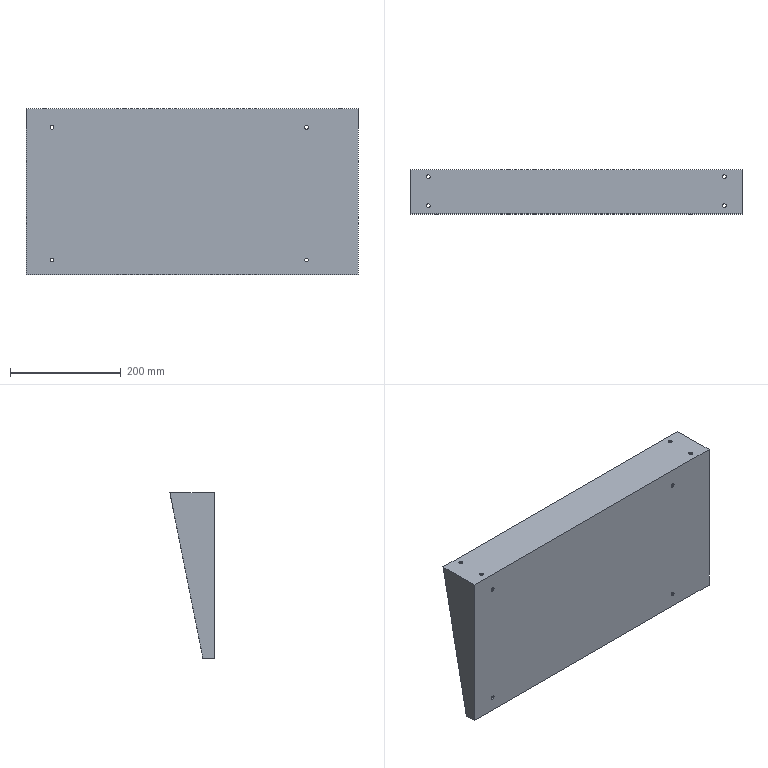Component | SolidWorks | OilTankBracket-1 | 1 solid | 26 faces | box 600 x 80 x 300 mm | volume 760356 mm3 | cylinder 16 | plane 10 | commonest cylinder face diameters 7 x16
build123d program:
from build123d import *

# Parameters (mm, degrees)
BOSS_EXTRUDE1_DEPTH = 600
SHELL1_T            = -3
SKETCH3_R           = 3.5
CUT_EXTRUDE1_DEPTH  = 3
LPATTERN1_COUNT     = 2
LPATTERN1_PITCH     = 535
SKETCH4_R           = 3.5
CUT_EXTRUDE2_DEPTH  = 3


with BuildPart() as part:
    # Sketch2 → Boss-Extrude1 (new body)
    with BuildSketch(Plane.XY):
        Polygon((17.897, -71.247), (17.897, 8.753), (317.897, 8.753), (317.897, -11.247), align=None)
    extrude(amount=BOSS_EXTRUDE1_DEPTH)

    # Shell1
    shell1_openings = [part.faces().sort_by_distance(p)[0] for p in [
        (317.897, -1.247, 300),
        (167.897, -41.247, 300),
    ]]
    offset(amount=SHELL1_T, openings=shell1_openings, kind=Kind.INTERSECTION)

    # Sketch3 → Cut-Extrude1 (cut)
    with BuildSketch(Plane(origin=(20.897, 0, 0), x_dir=(0, 0, -1), z_dir=(1, 0, 0))):
        with Locations((-567, -6.247)):
            Circle(SKETCH3_R)
        with Locations((-567, -58.647)):
            Circle(SKETCH3_R)
    cut_extrude1 = extrude(amount=-CUT_EXTRUDE1_DEPTH, mode=Mode.SUBTRACT)

    # LPattern1: Cut-Extrude1 ×2
    with Locations(*[(0, 0, -i * LPATTERN1_PITCH) for i in range(1, LPATTERN1_COUNT)]):
        add(cut_extrude1, mode=Mode.SUBTRACT)

    # Sketch4 → Cut-Extrude2 (cut)
    with BuildSketch(Plane(origin=(0, 5.753, 0), x_dir=(-1, 0, 0), z_dir=(0, -1, 0))):
        with Locations(Location((-290.897, -553, 0), (0, 0, 90))):
            Circle(SKETCH4_R)
        with Locations(Location((-50.897, -553, 0), (0, 0, 90))):
            Circle(SKETCH4_R)
        with Locations(Location((-290.897, -93, 0), (0, 0, 90))):
            Circle(SKETCH4_R)
        with Locations(Location((-50.897, -93, 0), (0, 0, 90))):
            Circle(SKETCH4_R)
    extrude(amount=-CUT_EXTRUDE2_DEPTH, mode=Mode.SUBTRACT)


solid = part.part

# Placed as in the assembly
solid = solid.moved(Location((508.45, -702.681, -350.622), (180, -90, 0)))
STEP:
#1=CARTESIAN_POINT('',(16.219,-28.009,-15.808));
#2=VERTEX_POINT('',#1);
#3=CARTESIAN_POINT('',(16.494,-28.009,-15.808));
#4=VERTEX_POINT('',#3);
#5=CARTESIAN_POINT('',(16.356,-28.009,-15.808));
#6=DIRECTION('',(0.,1.,0.));
#7=DIRECTION('',(1.,0.,0.));
#8=AXIS2_PLACEMENT_3D('',#5,#6,#7);
#9=CIRCLE('',#8,0.1378);
#10=EDGE_CURVE('',#2,#4,#9,.T.);
#11=ORIENTED_EDGE('',*,*,#10,.F.);
#12=CARTESIAN_POINT('',(16.219,-27.891,-15.808));
#13=VERTEX_POINT('',#12);
#14=CARTESIAN_POINT('',(16.219,-28.009,-15.808));
#15=DIRECTION('',(0.,1.,0.));
#16=VECTOR('',#15,39.37);
#17=LINE('',#14,#16);
#18=EDGE_CURVE('',#2,#13,#17,.T.);
#19=ORIENTED_EDGE('',*,*,#18,.T.);
#20=CARTESIAN_POINT('',(16.494,-27.891,-15.808));
#21=VERTEX_POINT('',#20);
#22=CARTESIAN_POINT('',(16.356,-27.891,-15.808));
#23=DIRECTION('',(0.,1.,0.));
#24=DIRECTION('',(1.,0.,0.));
#25=AXIS2_PLACEMENT_3D('',#22,#23,#24);
#26=CIRCLE('',#25,0.1378);
#27=EDGE_CURVE('',#13,#21,#26,.T.);
#28=ORIENTED_EDGE('',*,*,#27,.T.);
#29=CARTESIAN_POINT('',(16.494,-28.009,-15.808));
#30=DIRECTION('',(0.,1.,0.));
#31=VECTOR('',#30,39.37);
#32=LINE('',#29,#31);
#33=EDGE_CURVE('',#4,#21,#32,.T.);
#34=ORIENTED_EDGE('',*,*,#33,.F.);
#35=EDGE_LOOP('',(#11,#19,#28,#34));
#36=FACE_OUTER_BOUND('',#35,.T.);
#37=CARTESIAN_POINT('',(16.356,-28.009,-15.808));
#38=DIRECTION('',(0.,1.,0.));
#39=DIRECTION('',(1.,0.,0.));
#40=AXIS2_PLACEMENT_3D('',#37,#38,#39);
#41=CYLINDRICAL_SURFACE('',#40,0.1378);
#42=ADVANCED_FACE('',(#36),#41,.F.);
#43=CARTESIAN_POINT('',(16.219,-28.009,-25.257));
#44=VERTEX_POINT('',#43);
#45=CARTESIAN_POINT('',(16.494,-28.009,-25.257));
#46=VERTEX_POINT('',#45);
#47=CARTESIAN_POINT('',(16.356,-28.009,-25.257));
#48=DIRECTION('',(0.,1.,0.));
#49=DIRECTION('',(1.,0.,0.));
#50=AXIS2_PLACEMENT_3D('',#47,#48,#49);
#51=CIRCLE('',#50,0.1378);
#52=EDGE_CURVE('',#44,#46,#51,.T.);
#53=ORIENTED_EDGE('',*,*,#52,.F.);
#54=CARTESIAN_POINT('',(16.219,-27.891,-25.257));
#55=VERTEX_POINT('',#54);
#56=CARTESIAN_POINT('',(16.219,-28.009,-25.257));
#57=DIRECTION('',(0.,1.,0.));
#58=VECTOR('',#57,39.37);
#59=LINE('',#56,#58);
#60=EDGE_CURVE('',#44,#55,#59,.T.);
#61=ORIENTED_EDGE('',*,*,#60,.T.);
#62=CARTESIAN_POINT('',(16.494,-27.891,-25.257));
#63=VERTEX_POINT('',#62);
#64=CARTESIAN_POINT('',(16.356,-27.891,-25.257));
#65=DIRECTION('',(0.,1.,0.));
#66=DIRECTION('',(1.,0.,0.));
#67=AXIS2_PLACEMENT_3D('',#64,#65,#66);
#68=CIRCLE('',#67,0.1378);
#69=EDGE_CURVE('',#55,#63,#68,.T.);
#70=ORIENTED_EDGE('',*,*,#69,.T.);
#71=CARTESIAN_POINT('',(16.494,-28.009,-25.257));
#72=DIRECTION('',(0.,1.,0.));
#73=VECTOR('',#72,39.37);
#74=LINE('',#71,#73);
#75=EDGE_CURVE('',#46,#63,#74,.T.);
#76=ORIENTED_EDGE('',*,*,#75,.F.);
#77=EDGE_LOOP('',(#53,#61,#70,#76));
#78=FACE_OUTER_BOUND('',#77,.T.);
#79=CARTESIAN_POINT('',(16.356,-28.009,-25.257));
#80=DIRECTION('',(0.,1.,0.));
#81=DIRECTION('',(1.,0.,0.));
#82=AXIS2_PLACEMENT_3D('',#79,#80,#81);
#83=CYLINDRICAL_SURFACE('',#82,0.1378);
#84=ADVANCED_FACE('',(#78),#83,.F.);
#85=CARTESIAN_POINT('',(-1.892,-28.009,-15.808));
#86=VERTEX_POINT('',#85);
#87=CARTESIAN_POINT('',(-1.616,-28.009,-15.808));
#88=VERTEX_POINT('',#87);
#89=CARTESIAN_POINT('',(-1.754,-28.009,-15.808));
#90=DIRECTION('',(0.,1.,0.));
#91=DIRECTION('',(1.,0.,0.));
#92=AXIS2_PLACEMENT_3D('',#89,#90,#91);
#93=CIRCLE('',#92,0.1378);
#94=EDGE_CURVE('',#86,#88,#93,.T.);
#95=ORIENTED_EDGE('',*,*,#94,.F.);
#96=CARTESIAN_POINT('',(-1.892,-27.891,-15.808));
#97=VERTEX_POINT('',#96);
#98=CARTESIAN_POINT('',(-1.892,-28.009,-15.808));
#99=DIRECTION('',(0.,1.,0.));
#100=VECTOR('',#99,39.37);
#101=LINE('',#98,#100);
#102=EDGE_CURVE('',#86,#97,#101,.T.);
#103=ORIENTED_EDGE('',*,*,#102,.T.);
#104=CARTESIAN_POINT('',(-1.616,-27.891,-15.808));
#105=VERTEX_POINT('',#104);
#106=CARTESIAN_POINT('',(-1.754,-27.891,-15.808));
#107=DIRECTION('',(0.,1.,0.));
#108=DIRECTION('',(1.,0.,0.));
#109=AXIS2_PLACEMENT_3D('',#106,#107,#108);
#110=CIRCLE('',#109,0.1378);
#111=EDGE_CURVE('',#97,#105,#110,.T.);
#112=ORIENTED_EDGE('',*,*,#111,.T.);
#113=CARTESIAN_POINT('',(-1.616,-28.009,-15.808));
#114=DIRECTION('',(0.,1.,0.));
#115=VECTOR('',#114,39.37);
#116=LINE('',#113,#115);
#117=EDGE_CURVE('',#88,#105,#116,.T.);
#118=ORIENTED_EDGE('',*,*,#117,.F.);
#119=EDGE_LOOP('',(#95,#103,#112,#118));
#120=FACE_OUTER_BOUND('',#119,.T.);
#121=CARTESIAN_POINT('',(-1.754,-28.009,-15.808));
#122=DIRECTION('',(0.,1.,0.));
#123=DIRECTION('',(1.,0.,0.));
#124=AXIS2_PLACEMENT_3D('',#121,#122,#123);
#125=CYLINDRICAL_SURFACE('',#124,0.1378);
#126=ADVANCED_FACE('',(#120),#125,.F.);
#127=CARTESIAN_POINT('',(-1.892,-28.009,-25.257));
#128=VERTEX_POINT('',#127);
#129=CARTESIAN_POINT('',(-1.616,-28.009,-25.257));
#130=VERTEX_POINT('',#129);
#131=CARTESIAN_POINT('',(-1.754,-28.009,-25.257));
#132=DIRECTION('',(0.,1.,0.));
#133=DIRECTION('',(1.,0.,0.));
#134=AXIS2_PLACEMENT_3D('',#131,#132,#133);
#135=CIRCLE('',#134,0.1378);
#136=EDGE_CURVE('',#128,#130,#135,.T.);
#137=ORIENTED_EDGE('',*,*,#136,.F.);
#138=CARTESIAN_POINT('',(-1.892,-27.891,-25.257));
#139=VERTEX_POINT('',#138);
#140=CARTESIAN_POINT('',(-1.892,-28.009,-25.257));
#141=DIRECTION('',(0.,1.,0.));
#142=VECTOR('',#141,39.37);
#143=LINE('',#140,#142);
#144=EDGE_CURVE('',#128,#139,#143,.T.);
#145=ORIENTED_EDGE('',*,*,#144,.T.);
#146=CARTESIAN_POINT('',(-1.616,-27.891,-25.257));
#147=VERTEX_POINT('',#146);
#148=CARTESIAN_POINT('',(-1.754,-27.891,-25.257));
#149=DIRECTION('',(0.,1.,0.));
#150=DIRECTION('',(1.,0.,0.));
#151=AXIS2_PLACEMENT_3D('',#148,#149,#150);
#152=CIRCLE('',#151,0.1378);
#153=EDGE_CURVE('',#139,#147,#152,.T.);
#154=ORIENTED_EDGE('',*,*,#153,.T.);
#155=CARTESIAN_POINT('',(-1.616,-28.009,-25.257));
#156=DIRECTION('',(0.,1.,0.));
#157=VECTOR('',#156,39.37);
#158=LINE('',#155,#157);
#159=EDGE_CURVE('',#130,#147,#158,.T.);
#160=ORIENTED_EDGE('',*,*,#159,.F.);
#161=EDGE_LOOP('',(#137,#145,#154,#160));
#162=FACE_OUTER_BOUND('',#161,.T.);
#163=CARTESIAN_POINT('',(-1.754,-28.009,-25.257));
#164=DIRECTION('',(0.,1.,0.));
#165=DIRECTION('',(1.,0.,0.));
#166=AXIS2_PLACEMENT_3D('',#163,#164,#165);
#167=CYLINDRICAL_SURFACE('',#166,0.1378);
#168=ADVANCED_FACE('',(#162),#167,.F.);
#169=CARTESIAN_POINT('',(18.62,-25.356,-14.509));
#170=VERTEX_POINT('',#169);
#171=CARTESIAN_POINT('',(18.896,-25.356,-14.509));
#172=VERTEX_POINT('',#171);
#173=CARTESIAN_POINT('',(18.758,-25.356,-14.509));
#174=DIRECTION('',(-0.,0.,-1.));
#175=DIRECTION('',(1.,0.,0.));
#176=AXIS2_PLACEMENT_3D('',#173,#174,#175);
#177=CIRCLE('',#176,0.1378);
#178=EDGE_CURVE('',#170,#172,#177,.T.);
#179=ORIENTED_EDGE('',*,*,#178,.F.);
#180=CARTESIAN_POINT('',(18.62,-25.356,-14.627));
#181=VERTEX_POINT('',#180);
#182=CARTESIAN_POINT('',(18.62,-25.356,-14.509));
#183=DIRECTION('',(-0.,0.,-1.));
#184=VECTOR('',#183,39.37);
#185=LINE('',#182,#184);
#186=EDGE_CURVE('',#170,#181,#185,.T.);
#187=ORIENTED_EDGE('',*,*,#186,.T.);
#188=CARTESIAN_POINT('',(18.896,-25.356,-14.627));
#189=VERTEX_POINT('',#188);
#190=CARTESIAN_POINT('',(18.758,-25.356,-14.627));
#191=DIRECTION('',(-0.,0.,-1.));
#192=DIRECTION('',(1.,0.,0.));
#193=AXIS2_PLACEMENT_3D('',#190,#191,#192);
#194=CIRCLE('',#193,0.1378);
#195=EDGE_CURVE('',#181,#189,#194,.T.);
#196=ORIENTED_EDGE('',*,*,#195,.T.);
#197=CARTESIAN_POINT('',(18.896,-25.356,-14.509));
#198=DIRECTION('',(-0.,0.,-1.));
#199=VECTOR('',#198,39.37);
#200=LINE('',#197,#199);
#201=EDGE_CURVE('',#172,#189,#200,.T.);
#202=ORIENTED_EDGE('',*,*,#201,.F.);
#203=EDGE_LOOP('',(#179,#187,#196,#202));
#204=FACE_OUTER_BOUND('',#203,.T.);
#205=CARTESIAN_POINT('',(18.758,-25.356,-14.509));
#206=DIRECTION('',(-0.,0.,-1.));
#207=DIRECTION('',(1.,0.,0.));
#208=AXIS2_PLACEMENT_3D('',#205,#206,#207);
#209=CYLINDRICAL_SURFACE('',#208,0.1378);
#210=ADVANCED_FACE('',(#204),#209,.F.);
#211=CARTESIAN_POINT('',(18.62,-27.419,-14.509));
#212=VERTEX_POINT('',#211);
#213=CARTESIAN_POINT('',(18.896,-27.419,-14.509));
#214=VERTEX_POINT('',#213);
#215=CARTESIAN_POINT('',(18.758,-27.419,-14.509));
#216=DIRECTION('',(-0.,0.,-1.));
#217=DIRECTION('',(1.,0.,0.));
#218=AXIS2_PLACEMENT_3D('',#215,#216,#217);
#219=CIRCLE('',#218,0.1378);
#220=EDGE_CURVE('',#212,#214,#219,.T.);
#221=ORIENTED_EDGE('',*,*,#220,.F.);
#222=CARTESIAN_POINT('',(18.62,-27.419,-14.627));
#223=VERTEX_POINT('',#222);
#224=CARTESIAN_POINT('',(18.62,-27.419,-14.509));
#225=DIRECTION('',(-0.,0.,-1.));
#226=VECTOR('',#225,39.37);
#227=LINE('',#224,#226);
#228=EDGE_CURVE('',#212,#223,#227,.T.);
#229=ORIENTED_EDGE('',*,*,#228,.T.);
#230=CARTESIAN_POINT('',(18.896,-27.419,-14.627));
#231=VERTEX_POINT('',#230);
#232=CARTESIAN_POINT('',(18.758,-27.419,-14.627));
#233=DIRECTION('',(-0.,0.,-1.));
#234=DIRECTION('',(1.,0.,0.));
#235=AXIS2_PLACEMENT_3D('',#232,#233,#234);
#236=CIRCLE('',#235,0.1378);
#237=EDGE_CURVE('',#223,#231,#236,.T.);
#238=ORIENTED_EDGE('',*,*,#237,.T.);
#239=CARTESIAN_POINT('',(18.896,-27.419,-14.509));
#240=DIRECTION('',(-0.,0.,-1.));
#241=VECTOR('',#240,39.37);
#242=LINE('',#239,#241);
#243=EDGE_CURVE('',#214,#231,#242,.T.);
#244=ORIENTED_EDGE('',*,*,#243,.F.);
#245=EDGE_LOOP('',(#221,#229,#238,#244));
#246=FACE_OUTER_BOUND('',#245,.T.);
#247=CARTESIAN_POINT('',(18.758,-27.419,-14.509));
#248=DIRECTION('',(-0.,0.,-1.));
#249=DIRECTION('',(1.,0.,0.));
#250=AXIS2_PLACEMENT_3D('',#247,#248,#249);
#251=CYLINDRICAL_SURFACE('',#250,0.1378);
#252=ADVANCED_FACE('',(#246),#251,.F.);
#253=CARTESIAN_POINT('',(-2.443,-25.356,-14.509));
#254=VERTEX_POINT('',#253);
#255=CARTESIAN_POINT('',(-2.167,-25.356,-14.509));
#256=VERTEX_POINT('',#255);
#257=CARTESIAN_POINT('',(-2.305,-25.356,-14.509));
#258=DIRECTION('',(-0.,0.,-1.));
#259=DIRECTION('',(1.,0.,0.));
#260=AXIS2_PLACEMENT_3D('',#257,#258,#259);
#261=CIRCLE('',#260,0.1378);
#262=EDGE_CURVE('',#254,#256,#261,.T.);
#263=ORIENTED_EDGE('',*,*,#262,.F.);
#264=CARTESIAN_POINT('',(-2.443,-25.356,-14.627));
#265=VERTEX_POINT('',#264);
#266=CARTESIAN_POINT('',(-2.443,-25.356,-14.509));
#267=DIRECTION('',(-0.,0.,-1.));
#268=VECTOR('',#267,39.37);
#269=LINE('',#266,#268);
#270=EDGE_CURVE('',#254,#265,#269,.T.);
#271=ORIENTED_EDGE('',*,*,#270,.T.);
#272=CARTESIAN_POINT('',(-2.167,-25.356,-14.627));
#273=VERTEX_POINT('',#272);
#274=CARTESIAN_POINT('',(-2.305,-25.356,-14.627));
#275=DIRECTION('',(-0.,0.,-1.));
#276=DIRECTION('',(1.,0.,0.));
#277=AXIS2_PLACEMENT_3D('',#274,#275,#276);
#278=CIRCLE('',#277,0.1378);
#279=EDGE_CURVE('',#265,#273,#278,.T.);
#280=ORIENTED_EDGE('',*,*,#279,.T.);
#281=CARTESIAN_POINT('',(-2.167,-25.356,-14.509));
#282=DIRECTION('',(-0.,0.,-1.));
#283=VECTOR('',#282,39.37);
#284=LINE('',#281,#283);
#285=EDGE_CURVE('',#256,#273,#284,.T.);
#286=ORIENTED_EDGE('',*,*,#285,.F.);
#287=EDGE_LOOP('',(#263,#271,#280,#286));
#288=FACE_OUTER_BOUND('',#287,.T.);
#289=CARTESIAN_POINT('',(-2.305,-25.356,-14.509));
#290=DIRECTION('',(-0.,0.,-1.));
#291=DIRECTION('',(1.,0.,0.));
#292=AXIS2_PLACEMENT_3D('',#289,#290,#291);
#293=CYLINDRICAL_SURFACE('',#292,0.1378);
#294=ADVANCED_FACE('',(#288),#293,.F.);
#295=CARTESIAN_POINT('',(-2.443,-27.419,-14.509));
#296=VERTEX_POINT('',#295);
#297=CARTESIAN_POINT('',(-2.167,-27.419,-14.509));
#298=VERTEX_POINT('',#297);
#299=CARTESIAN_POINT('',(-2.305,-27.419,-14.509));
#300=DIRECTION('',(-0.,0.,-1.));
#301=DIRECTION('',(1.,0.,0.));
#302=AXIS2_PLACEMENT_3D('',#299,#300,#301);
#303=CIRCLE('',#302,0.1378);
#304=EDGE_CURVE('',#296,#298,#303,.T.);
#305=ORIENTED_EDGE('',*,*,#304,.F.);
#306=CARTESIAN_POINT('',(-2.443,-27.419,-14.627));
#307=VERTEX_POINT('',#306);
#308=CARTESIAN_POINT('',(-2.443,-27.419,-14.509));
#309=DIRECTION('',(-0.,0.,-1.));
#310=VECTOR('',#309,39.37);
#311=LINE('',#308,#310);
#312=EDGE_CURVE('',#296,#307,#311,.T.);
#313=ORIENTED_EDGE('',*,*,#312,.T.);
#314=CARTESIAN_POINT('',(-2.167,-27.419,-14.627));
#315=VERTEX_POINT('',#314);
#316=CARTESIAN_POINT('',(-2.305,-27.419,-14.627));
#317=DIRECTION('',(-0.,0.,-1.));
#318=DIRECTION('',(1.,0.,0.));
#319=AXIS2_PLACEMENT_3D('',#316,#317,#318);
#320=CIRCLE('',#319,0.1378);
#321=EDGE_CURVE('',#307,#315,#320,.T.);
#322=ORIENTED_EDGE('',*,*,#321,.T.);
#323=CARTESIAN_POINT('',(-2.167,-27.419,-14.509));
#324=DIRECTION('',(-0.,0.,-1.));
#325=VECTOR('',#324,39.37);
#326=LINE('',#323,#325);
#327=EDGE_CURVE('',#298,#315,#326,.T.);
#328=ORIENTED_EDGE('',*,*,#327,.F.);
#329=EDGE_LOOP('',(#305,#313,#322,#328));
#330=FACE_OUTER_BOUND('',#329,.T.);
#331=CARTESIAN_POINT('',(-2.305,-27.419,-14.509));
#332=DIRECTION('',(-0.,0.,-1.));
#333=DIRECTION('',(1.,0.,0.));
#334=AXIS2_PLACEMENT_3D('',#331,#332,#333);
#335=CYLINDRICAL_SURFACE('',#334,0.1378);
#336=ADVANCED_FACE('',(#330),#335,.F.);
#337=CARTESIAN_POINT('',(19.9,-24.883,-14.627));
#338=VERTEX_POINT('',#337);
#339=CARTESIAN_POINT('',(19.9,-27.222,-26.32));
#340=VERTEX_POINT('',#339);
#341=CARTESIAN_POINT('',(19.9,-24.832,-14.371));
#342=DIRECTION('',(-0.,-0.1961,-0.9806));
#343=VECTOR('',#342,39.37);
#344=LINE('',#341,#343);
#345=EDGE_CURVE('',#338,#340,#344,.T.);
#346=ORIENTED_EDGE('',*,*,#345,.F.);
#347=CARTESIAN_POINT('',(-3.486,-24.883,-14.627));
#348=VERTEX_POINT('',#347);
#349=CARTESIAN_POINT('',(-3.604,-24.883,-14.627));
#350=DIRECTION('',(1.,-0.,-0.));
#351=VECTOR('',#350,39.37);
#352=LINE('',#349,#351);
#353=EDGE_CURVE('',#348,#338,#352,.T.);
#354=ORIENTED_EDGE('',*,*,#353,.F.);
#355=CARTESIAN_POINT('',(-3.486,-27.222,-26.32));
#356=VERTEX_POINT('',#355);
#357=CARTESIAN_POINT('',(-3.486,-24.832,-14.371));
#358=DIRECTION('',(-0.,-0.1961,-0.9806));
#359=VECTOR('',#358,39.37);
#360=LINE('',#357,#359);
#361=EDGE_CURVE('',#348,#356,#360,.T.);
#362=ORIENTED_EDGE('',*,*,#361,.T.);
#363=CARTESIAN_POINT('',(-3.604,-27.222,-26.32));
#364=VERTEX_POINT('',#363);
#365=CARTESIAN_POINT('',(-3.604,-27.222,-26.32));
#366=DIRECTION('',(1.,-0.,-0.));
#367=VECTOR('',#366,39.37);
#368=LINE('',#365,#367);
#369=EDGE_CURVE('',#364,#356,#368,.T.);
#370=ORIENTED_EDGE('',*,*,#369,.F.);
#371=CARTESIAN_POINT('',(-3.604,-24.86,-14.509));
#372=VERTEX_POINT('',#371);
#373=CARTESIAN_POINT('',(-3.604,-27.222,-26.32));
#374=DIRECTION('',(-0.,-0.1961,-0.9806));
#375=VECTOR('',#374,39.37);
#376=LINE('',#373,#375);
#377=EDGE_CURVE('',#372,#364,#376,.T.);
#378=ORIENTED_EDGE('',*,*,#377,.F.);
#379=CARTESIAN_POINT('',(20.018,-24.86,-14.509));
#380=VERTEX_POINT('',#379);
#381=CARTESIAN_POINT('',(-3.604,-24.86,-14.509));
#382=DIRECTION('',(1.,-0.,-0.));
#383=VECTOR('',#382,39.37);
#384=LINE('',#381,#383);
#385=EDGE_CURVE('',#372,#380,#384,.T.);
#386=ORIENTED_EDGE('',*,*,#385,.T.);
#387=CARTESIAN_POINT('',(20.018,-27.222,-26.32));
#388=VERTEX_POINT('',#387);
#389=CARTESIAN_POINT('',(20.018,-27.222,-26.32));
#390=DIRECTION('',(-0.,-0.1961,-0.9806));
#391=VECTOR('',#390,39.37);
#392=LINE('',#389,#391);
#393=EDGE_CURVE('',#380,#388,#392,.T.);
#394=ORIENTED_EDGE('',*,*,#393,.T.);
#395=CARTESIAN_POINT('',(-3.604,-27.222,-26.32));
#396=DIRECTION('',(1.,-0.,-0.));
#397=VECTOR('',#396,39.37);
#398=LINE('',#395,#397);
#399=EDGE_CURVE('',#340,#388,#398,.T.);
#400=ORIENTED_EDGE('',*,*,#399,.F.);
#401=EDGE_LOOP('',(#346,#354,#362,#370,#378,#386,#394,#400));
#402=FACE_OUTER_BOUND('',#401,.T.);
#403=CARTESIAN_POINT('',(-3.604,-27.222,-26.32));
#404=DIRECTION('',(-0.,-0.9806,0.1961));
#405=DIRECTION('',(0.,0.1961,0.9806));
#406=AXIS2_PLACEMENT_3D('',#403,#404,#405);
#407=PLANE('',#406);
#408=ADVANCED_FACE('',(#402),#407,.F.);
#409=CARTESIAN_POINT('',(19.9,-27.891,-26.32));
#410=VERTEX_POINT('',#409);
#411=CARTESIAN_POINT('',(19.9,-27.665,-26.32));
#412=DIRECTION('',(-0.,-1.,-0.));
#413=VECTOR('',#412,39.37);
#414=LINE('',#411,#413);
#415=EDGE_CURVE('',#340,#410,#414,.T.);
#416=ORIENTED_EDGE('',*,*,#415,.F.);
#417=ORIENTED_EDGE('',*,*,#399,.T.);
#418=CARTESIAN_POINT('',(20.018,-28.009,-26.32));
#419=VERTEX_POINT('',#418);
#420=CARTESIAN_POINT('',(20.018,-28.009,-26.32));
#421=DIRECTION('',(-0.,-1.,-0.));
#422=VECTOR('',#421,39.37);
#423=LINE('',#420,#422);
#424=EDGE_CURVE('',#388,#419,#423,.T.);
#425=ORIENTED_EDGE('',*,*,#424,.T.);
#426=CARTESIAN_POINT('',(-3.604,-28.009,-26.32));
#427=VERTEX_POINT('',#426);
#428=CARTESIAN_POINT('',(-3.604,-28.009,-26.32));
#429=DIRECTION('',(1.,-0.,-0.));
#430=VECTOR('',#429,39.37);
#431=LINE('',#428,#430);
#432=EDGE_CURVE('',#427,#419,#431,.T.);
#433=ORIENTED_EDGE('',*,*,#432,.F.);
#434=CARTESIAN_POINT('',(-3.604,-28.009,-26.32));
#435=DIRECTION('',(-0.,-1.,-0.));
#436=VECTOR('',#435,39.37);
#437=LINE('',#434,#436);
#438=EDGE_CURVE('',#364,#427,#437,.T.);
#439=ORIENTED_EDGE('',*,*,#438,.F.);
#440=ORIENTED_EDGE('',*,*,#369,.T.);
#441=CARTESIAN_POINT('',(-3.486,-27.891,-26.32));
#442=VERTEX_POINT('',#441);
#443=CARTESIAN_POINT('',(-3.486,-27.665,-26.32));
#444=DIRECTION('',(-0.,-1.,-0.));
#445=VECTOR('',#444,39.37);
#446=LINE('',#443,#445);
#447=EDGE_CURVE('',#356,#442,#446,.T.);
#448=ORIENTED_EDGE('',*,*,#447,.T.);
#449=CARTESIAN_POINT('',(-3.604,-27.891,-26.32));
#450=DIRECTION('',(1.,-0.,-0.));
#451=VECTOR('',#450,39.37);
#452=LINE('',#449,#451);
#453=EDGE_CURVE('',#442,#410,#452,.T.);
#454=ORIENTED_EDGE('',*,*,#453,.T.);
#455=EDGE_LOOP('',(#416,#417,#425,#433,#439,#440,#448,#454));
#456=FACE_OUTER_BOUND('',#455,.T.);
#457=CARTESIAN_POINT('',(-3.604,-28.009,-26.32));
#458=DIRECTION('',(0.,-0.,1.));
#459=DIRECTION('',(-1.,0.,0.));
#460=AXIS2_PLACEMENT_3D('',#457,#458,#459);
#461=PLANE('',#460);
#462=ADVANCED_FACE('',(#456),#461,.F.);
#463=CARTESIAN_POINT('',(16.356,-28.009,-15.808));
#464=DIRECTION('',(0.,1.,0.));
#465=DIRECTION('',(1.,0.,0.));
#466=AXIS2_PLACEMENT_3D('',#463,#464,#465);
#467=CIRCLE('',#466,0.1378);
#468=EDGE_CURVE('',#4,#2,#467,.T.);
#469=ORIENTED_EDGE('',*,*,#468,.T.);
#470=ORIENTED_EDGE('',*,*,#10,.T.);
#471=EDGE_LOOP('',(#469,#470));
#472=FACE_BOUND('',#471,.T.);
#473=CARTESIAN_POINT('',(16.356,-28.009,-25.257));
#474=DIRECTION('',(0.,1.,0.));
#475=DIRECTION('',(1.,0.,0.));
#476=AXIS2_PLACEMENT_3D('',#473,#474,#475);
#477=CIRCLE('',#476,0.1378);
#478=EDGE_CURVE('',#46,#44,#477,.T.);
#479=ORIENTED_EDGE('',*,*,#478,.T.);
#480=ORIENTED_EDGE('',*,*,#52,.T.);
#481=EDGE_LOOP('',(#479,#480));
#482=FACE_BOUND('',#481,.T.);
#483=CARTESIAN_POINT('',(-1.754,-28.009,-15.808));
#484=DIRECTION('',(0.,1.,0.));
#485=DIRECTION('',(1.,0.,0.));
#486=AXIS2_PLACEMENT_3D('',#483,#484,#485);
#487=CIRCLE('',#486,0.1378);
#488=EDGE_CURVE('',#88,#86,#487,.T.);
#489=ORIENTED_EDGE('',*,*,#488,.T.);
#490=ORIENTED_EDGE('',*,*,#94,.T.);
#491=EDGE_LOOP('',(#489,#490));
#492=FACE_BOUND('',#491,.T.);
#493=CARTESIAN_POINT('',(-1.754,-28.009,-25.257));
#494=DIRECTION('',(0.,1.,0.));
#495=DIRECTION('',(1.,0.,0.));
#496=AXIS2_PLACEMENT_3D('',#493,#494,#495);
#497=CIRCLE('',#496,0.1378);
#498=EDGE_CURVE('',#130,#128,#497,.T.);
#499=ORIENTED_EDGE('',*,*,#498,.T.);
#500=ORIENTED_EDGE('',*,*,#136,.T.);
#501=EDGE_LOOP('',(#499,#500));
#502=FACE_BOUND('',#501,.T.);
#503=CARTESIAN_POINT('',(20.018,-28.009,-14.509));
#504=VERTEX_POINT('',#503);
#505=CARTESIAN_POINT('',(20.018,-28.009,-14.509));
#506=DIRECTION('',(0.,-0.,1.));
#507=VECTOR('',#506,39.37);
#508=LINE('',#505,#507);
#509=EDGE_CURVE('',#419,#504,#508,.T.);
#510=ORIENTED_EDGE('',*,*,#509,.T.);
#511=CARTESIAN_POINT('',(-3.604,-28.009,-14.509));
#512=VERTEX_POINT('',#511);
#513=CARTESIAN_POINT('',(-3.604,-28.009,-14.509));
#514=DIRECTION('',(1.,-0.,-0.));
#515=VECTOR('',#514,39.37);
#516=LINE('',#513,#515);
#517=EDGE_CURVE('',#512,#504,#516,.T.);
#518=ORIENTED_EDGE('',*,*,#517,.F.);
#519=CARTESIAN_POINT('',(-3.604,-28.009,-14.509));
#520=DIRECTION('',(0.,-0.,1.));
#521=VECTOR('',#520,39.37);
#522=LINE('',#519,#521);
#523=EDGE_CURVE('',#427,#512,#522,.T.);
#524=ORIENTED_EDGE('',*,*,#523,.F.);
#525=ORIENTED_EDGE('',*,*,#432,.T.);
#526=EDGE_LOOP('',(#510,#518,#524,#525));
#527=FACE_OUTER_BOUND('',#526,.T.);
#528=CARTESIAN_POINT('',(-3.604,-28.009,-14.509));
#529=DIRECTION('',(0.,1.,0.));
#530=DIRECTION('',(1.,-0.,-0.));
#531=AXIS2_PLACEMENT_3D('',#528,#529,#530);
#532=PLANE('',#531);
#533=ADVANCED_FACE('',(#472,#482,#492,#502,#527),#532,.F.);
#534=CARTESIAN_POINT('',(18.758,-25.356,-14.509));
#535=DIRECTION('',(-0.,0.,-1.));
#536=DIRECTION('',(1.,0.,0.));
#537=AXIS2_PLACEMENT_3D('',#534,#535,#536);
#538=CIRCLE('',#537,0.1378);
#539=EDGE_CURVE('',#172,#170,#538,.T.);
#540=ORIENTED_EDGE('',*,*,#539,.T.);
#541=ORIENTED_EDGE('',*,*,#178,.T.);
#542=EDGE_LOOP('',(#540,#541));
#543=FACE_BOUND('',#542,.T.);
#544=CARTESIAN_POINT('',(18.758,-27.419,-14.509));
#545=DIRECTION('',(-0.,0.,-1.));
#546=DIRECTION('',(1.,0.,0.));
#547=AXIS2_PLACEMENT_3D('',#544,#545,#546);
#548=CIRCLE('',#547,0.1378);
#549=EDGE_CURVE('',#214,#212,#548,.T.);
#550=ORIENTED_EDGE('',*,*,#549,.T.);
#551=ORIENTED_EDGE('',*,*,#220,.T.);
#552=EDGE_LOOP('',(#550,#551));
#553=FACE_BOUND('',#552,.T.);
#554=CARTESIAN_POINT('',(-2.305,-25.356,-14.509));
#555=DIRECTION('',(-0.,0.,-1.));
#556=DIRECTION('',(1.,0.,0.));
#557=AXIS2_PLACEMENT_3D('',#554,#555,#556);
#558=CIRCLE('',#557,0.1378);
#559=EDGE_CURVE('',#256,#254,#558,.T.);
#560=ORIENTED_EDGE('',*,*,#559,.T.);
#561=ORIENTED_EDGE('',*,*,#262,.T.);
#562=EDGE_LOOP('',(#560,#561));
#563=FACE_BOUND('',#562,.T.);
#564=CARTESIAN_POINT('',(-2.305,-27.419,-14.509));
#565=DIRECTION('',(-0.,0.,-1.));
#566=DIRECTION('',(1.,0.,0.));
#567=AXIS2_PLACEMENT_3D('',#564,#565,#566);
#568=CIRCLE('',#567,0.1378);
#569=EDGE_CURVE('',#298,#296,#568,.T.);
#570=ORIENTED_EDGE('',*,*,#569,.T.);
#571=ORIENTED_EDGE('',*,*,#304,.T.);
#572=EDGE_LOOP('',(#570,#571));
#573=FACE_BOUND('',#572,.T.);
#574=CARTESIAN_POINT('',(20.018,-24.86,-14.509));
#575=DIRECTION('',(0.,1.,0.));
#576=VECTOR('',#575,39.37);
#577=LINE('',#574,#576);
#578=EDGE_CURVE('',#504,#380,#577,.T.);
#579=ORIENTED_EDGE('',*,*,#578,.T.);
#580=ORIENTED_EDGE('',*,*,#385,.F.);
#581=CARTESIAN_POINT('',(-3.604,-24.86,-14.509));
#582=DIRECTION('',(0.,1.,0.));
#583=VECTOR('',#582,39.37);
#584=LINE('',#581,#583);
#585=EDGE_CURVE('',#512,#372,#584,.T.);
#586=ORIENTED_EDGE('',*,*,#585,.F.);
#587=ORIENTED_EDGE('',*,*,#517,.T.);
#588=EDGE_LOOP('',(#579,#580,#586,#587));
#589=FACE_OUTER_BOUND('',#588,.T.);
#590=CARTESIAN_POINT('',(-3.604,-24.86,-14.509));
#591=DIRECTION('',(-0.,0.,-1.));
#592=DIRECTION('',(1.,-0.,-0.));
#593=AXIS2_PLACEMENT_3D('',#590,#591,#592);
#594=PLANE('',#593);
#595=ADVANCED_FACE('',(#543,#553,#563,#573,#589),#594,.F.);
#596=ORIENTED_EDGE('',*,*,#377,.T.);
#597=ORIENTED_EDGE('',*,*,#438,.T.);
#598=ORIENTED_EDGE('',*,*,#523,.T.);
#599=ORIENTED_EDGE('',*,*,#585,.T.);
#600=EDGE_LOOP('',(#596,#597,#598,#599));
#601=FACE_OUTER_BOUND('',#600,.T.);
#602=CARTESIAN_POINT('',(-3.604,-27.665,-13.804));
#603=DIRECTION('',(1.,-0.,-0.));
#604=DIRECTION('',(0.,-0.,1.));
#605=AXIS2_PLACEMENT_3D('',#602,#603,#604);
#606=PLANE('',#605);
#607=ADVANCED_FACE('',(#601),#606,.F.);
#608=ORIENTED_EDGE('',*,*,#393,.F.);
#609=ORIENTED_EDGE('',*,*,#578,.F.);
#610=ORIENTED_EDGE('',*,*,#509,.F.);
#611=ORIENTED_EDGE('',*,*,#424,.F.);
#612=EDGE_LOOP('',(#608,#609,#610,#611));
#613=FACE_OUTER_BOUND('',#612,.T.);
#614=CARTESIAN_POINT('',(20.018,-27.665,-13.804));
#615=DIRECTION('',(1.,-0.,-0.));
#616=DIRECTION('',(0.,-0.,1.));
#617=AXIS2_PLACEMENT_3D('',#614,#615,#616);
#618=PLANE('',#617);
#619=ADVANCED_FACE('',(#613),#618,.T.);
#620=CARTESIAN_POINT('',(16.356,-27.891,-15.808));
#621=DIRECTION('',(0.,1.,0.));
#622=DIRECTION('',(1.,0.,0.));
#623=AXIS2_PLACEMENT_3D('',#620,#621,#622);
#624=CIRCLE('',#623,0.1378);
#625=EDGE_CURVE('',#21,#13,#624,.T.);
#626=ORIENTED_EDGE('',*,*,#625,.F.);
#627=ORIENTED_EDGE('',*,*,#27,.F.);
#628=EDGE_LOOP('',(#626,#627));
#629=FACE_BOUND('',#628,.T.);
#630=CARTESIAN_POINT('',(16.356,-27.891,-25.257));
#631=DIRECTION('',(0.,1.,0.));
#632=DIRECTION('',(1.,0.,0.));
#633=AXIS2_PLACEMENT_3D('',#630,#631,#632);
#634=CIRCLE('',#633,0.1378);
#635=EDGE_CURVE('',#63,#55,#634,.T.);
#636=ORIENTED_EDGE('',*,*,#635,.F.);
#637=ORIENTED_EDGE('',*,*,#69,.F.);
#638=EDGE_LOOP('',(#636,#637));
#639=FACE_BOUND('',#638,.T.);
#640=CARTESIAN_POINT('',(-1.754,-27.891,-15.808));
#641=DIRECTION('',(0.,1.,0.));
#642=DIRECTION('',(1.,0.,0.));
#643=AXIS2_PLACEMENT_3D('',#640,#641,#642);
#644=CIRCLE('',#643,0.1378);
#645=EDGE_CURVE('',#105,#97,#644,.T.);
#646=ORIENTED_EDGE('',*,*,#645,.F.);
#647=ORIENTED_EDGE('',*,*,#111,.F.);
#648=EDGE_LOOP('',(#646,#647));
#649=FACE_BOUND('',#648,.T.);
#650=CARTESIAN_POINT('',(-1.754,-27.891,-25.257));
#651=DIRECTION('',(0.,1.,0.));
#652=DIRECTION('',(1.,0.,0.));
#653=AXIS2_PLACEMENT_3D('',#650,#651,#652);
#654=CIRCLE('',#653,0.1378);
#655=EDGE_CURVE('',#147,#139,#654,.T.);
#656=ORIENTED_EDGE('',*,*,#655,.F.);
#657=ORIENTED_EDGE('',*,*,#153,.F.);
#658=EDGE_LOOP('',(#656,#657));
#659=FACE_BOUND('',#658,.T.);
#660=CARTESIAN_POINT('',(19.9,-27.891,-14.627));
#661=VERTEX_POINT('',#660);
#662=CARTESIAN_POINT('',(19.9,-27.891,-13.804));
#663=DIRECTION('',(0.,-0.,1.));
#664=VECTOR('',#663,39.37);
#665=LINE('',#662,#664);
#666=EDGE_CURVE('',#410,#661,#665,.T.);
#667=ORIENTED_EDGE('',*,*,#666,.F.);
#668=ORIENTED_EDGE('',*,*,#453,.F.);
#669=CARTESIAN_POINT('',(-3.486,-27.891,-14.627));
#670=VERTEX_POINT('',#669);
#671=CARTESIAN_POINT('',(-3.486,-27.891,-13.804));
#672=DIRECTION('',(0.,-0.,1.));
#673=VECTOR('',#672,39.37);
#674=LINE('',#671,#673);
#675=EDGE_CURVE('',#442,#670,#674,.T.);
#676=ORIENTED_EDGE('',*,*,#675,.T.);
#677=CARTESIAN_POINT('',(-3.604,-27.891,-14.627));
#678=DIRECTION('',(1.,-0.,-0.));
#679=VECTOR('',#678,39.37);
#680=LINE('',#677,#679);
#681=EDGE_CURVE('',#670,#661,#680,.T.);
#682=ORIENTED_EDGE('',*,*,#681,.T.);
#683=EDGE_LOOP('',(#667,#668,#676,#682));
#684=FACE_OUTER_BOUND('',#683,.T.);
#685=CARTESIAN_POINT('',(-3.604,-27.891,-14.509));
#686=DIRECTION('',(0.,1.,0.));
#687=DIRECTION('',(1.,-0.,-0.));
#688=AXIS2_PLACEMENT_3D('',#685,#686,#687);
#689=PLANE('',#688);
#690=ADVANCED_FACE('',(#629,#639,#649,#659,#684),#689,.T.);
#691=CARTESIAN_POINT('',(18.758,-25.356,-14.627));
#692=DIRECTION('',(-0.,0.,-1.));
#693=DIRECTION('',(1.,0.,0.));
#694=AXIS2_PLACEMENT_3D('',#691,#692,#693);
#695=CIRCLE('',#694,0.1378);
#696=EDGE_CURVE('',#189,#181,#695,.T.);
#697=ORIENTED_EDGE('',*,*,#696,.F.);
#698=ORIENTED_EDGE('',*,*,#195,.F.);
#699=EDGE_LOOP('',(#697,#698));
#700=FACE_BOUND('',#699,.T.);
#701=CARTESIAN_POINT('',(18.758,-27.419,-14.627));
#702=DIRECTION('',(-0.,0.,-1.));
#703=DIRECTION('',(1.,0.,0.));
#704=AXIS2_PLACEMENT_3D('',#701,#702,#703);
#705=CIRCLE('',#704,0.1378);
#706=EDGE_CURVE('',#231,#223,#705,.T.);
#707=ORIENTED_EDGE('',*,*,#706,.F.);
#708=ORIENTED_EDGE('',*,*,#237,.F.);
#709=EDGE_LOOP('',(#707,#708));
#710=FACE_BOUND('',#709,.T.);
#711=CARTESIAN_POINT('',(-2.305,-25.356,-14.627));
#712=DIRECTION('',(-0.,0.,-1.));
#713=DIRECTION('',(1.,0.,0.));
#714=AXIS2_PLACEMENT_3D('',#711,#712,#713);
#715=CIRCLE('',#714,0.1378);
#716=EDGE_CURVE('',#273,#265,#715,.T.);
#717=ORIENTED_EDGE('',*,*,#716,.F.);
#718=ORIENTED_EDGE('',*,*,#279,.F.);
#719=EDGE_LOOP('',(#717,#718));
#720=FACE_BOUND('',#719,.T.);
#721=CARTESIAN_POINT('',(-2.305,-27.419,-14.627));
#722=DIRECTION('',(-0.,0.,-1.));
#723=DIRECTION('',(1.,0.,0.));
#724=AXIS2_PLACEMENT_3D('',#721,#722,#723);
#725=CIRCLE('',#724,0.1378);
#726=EDGE_CURVE('',#315,#307,#725,.T.);
#727=ORIENTED_EDGE('',*,*,#726,.F.);
#728=ORIENTED_EDGE('',*,*,#321,.F.);
#729=EDGE_LOOP('',(#727,#728));
#730=FACE_BOUND('',#729,.T.);
#731=CARTESIAN_POINT('',(19.9,-27.665,-14.627));
#732=DIRECTION('',(0.,1.,0.));
#733=VECTOR('',#732,39.37);
#734=LINE('',#731,#733);
#735=EDGE_CURVE('',#661,#338,#734,.T.);
#736=ORIENTED_EDGE('',*,*,#735,.F.);
#737=ORIENTED_EDGE('',*,*,#681,.F.);
#738=CARTESIAN_POINT('',(-3.486,-27.665,-14.627));
#739=DIRECTION('',(0.,1.,0.));
#740=VECTOR('',#739,39.37);
#741=LINE('',#738,#740);
#742=EDGE_CURVE('',#670,#348,#741,.T.);
#743=ORIENTED_EDGE('',*,*,#742,.T.);
#744=ORIENTED_EDGE('',*,*,#353,.T.);
#745=EDGE_LOOP('',(#736,#737,#743,#744));
#746=FACE_OUTER_BOUND('',#745,.T.);
#747=CARTESIAN_POINT('',(-3.604,-24.86,-14.627));
#748=DIRECTION('',(-0.,0.,-1.));
#749=DIRECTION('',(1.,-0.,-0.));
#750=AXIS2_PLACEMENT_3D('',#747,#748,#749);
#751=PLANE('',#750);
#752=ADVANCED_FACE('',(#700,#710,#720,#730,#746),#751,.T.);
#753=ORIENTED_EDGE('',*,*,#361,.F.);
#754=ORIENTED_EDGE('',*,*,#742,.F.);
#755=ORIENTED_EDGE('',*,*,#675,.F.);
#756=ORIENTED_EDGE('',*,*,#447,.F.);
#757=EDGE_LOOP('',(#753,#754,#755,#756));
#758=FACE_OUTER_BOUND('',#757,.T.);
#759=CARTESIAN_POINT('',(-3.486,-27.665,-13.804));
#760=DIRECTION('',(1.,-0.,-0.));
#761=DIRECTION('',(0.,-0.,1.));
#762=AXIS2_PLACEMENT_3D('',#759,#760,#761);
#763=PLANE('',#762);
#764=ADVANCED_FACE('',(#758),#763,.T.);
#765=ORIENTED_EDGE('',*,*,#345,.T.);
#766=ORIENTED_EDGE('',*,*,#415,.T.);
#767=ORIENTED_EDGE('',*,*,#666,.T.);
#768=ORIENTED_EDGE('',*,*,#735,.T.);
#769=EDGE_LOOP('',(#765,#766,#767,#768));
#770=FACE_OUTER_BOUND('',#769,.T.);
#771=CARTESIAN_POINT('',(19.9,-27.665,-13.804));
#772=DIRECTION('',(1.,-0.,-0.));
#773=DIRECTION('',(0.,-0.,1.));
#774=AXIS2_PLACEMENT_3D('',#771,#772,#773);
#775=PLANE('',#774);
#776=ADVANCED_FACE('',(#770),#775,.F.);
#777=ORIENTED_EDGE('',*,*,#312,.F.);
#778=ORIENTED_EDGE('',*,*,#569,.F.);
#779=ORIENTED_EDGE('',*,*,#327,.T.);
#780=ORIENTED_EDGE('',*,*,#726,.T.);
#781=EDGE_LOOP('',(#777,#778,#779,#780));
#782=FACE_OUTER_BOUND('',#781,.T.);
#783=CARTESIAN_POINT('',(-2.305,-27.419,-14.509));
#784=DIRECTION('',(-0.,0.,-1.));
#785=DIRECTION('',(1.,0.,0.));
#786=AXIS2_PLACEMENT_3D('',#783,#784,#785);
#787=CYLINDRICAL_SURFACE('',#786,0.1378);
#788=ADVANCED_FACE('',(#782),#787,.F.);
#789=ORIENTED_EDGE('',*,*,#270,.F.);
#790=ORIENTED_EDGE('',*,*,#559,.F.);
#791=ORIENTED_EDGE('',*,*,#285,.T.);
#792=ORIENTED_EDGE('',*,*,#716,.T.);
#793=EDGE_LOOP('',(#789,#790,#791,#792));
#794=FACE_OUTER_BOUND('',#793,.T.);
#795=CARTESIAN_POINT('',(-2.305,-25.356,-14.509));
#796=DIRECTION('',(-0.,0.,-1.));
#797=DIRECTION('',(1.,0.,0.));
#798=AXIS2_PLACEMENT_3D('',#795,#796,#797);
#799=CYLINDRICAL_SURFACE('',#798,0.1378);
#800=ADVANCED_FACE('',(#794),#799,.F.);
#801=ORIENTED_EDGE('',*,*,#228,.F.);
#802=ORIENTED_EDGE('',*,*,#549,.F.);
#803=ORIENTED_EDGE('',*,*,#243,.T.);
#804=ORIENTED_EDGE('',*,*,#706,.T.);
#805=EDGE_LOOP('',(#801,#802,#803,#804));
#806=FACE_OUTER_BOUND('',#805,.T.);
#807=CARTESIAN_POINT('',(18.758,-27.419,-14.509));
#808=DIRECTION('',(-0.,0.,-1.));
#809=DIRECTION('',(1.,0.,0.));
#810=AXIS2_PLACEMENT_3D('',#807,#808,#809);
#811=CYLINDRICAL_SURFACE('',#810,0.1378);
#812=ADVANCED_FACE('',(#806),#811,.F.);
#813=ORIENTED_EDGE('',*,*,#186,.F.);
#814=ORIENTED_EDGE('',*,*,#539,.F.);
#815=ORIENTED_EDGE('',*,*,#201,.T.);
#816=ORIENTED_EDGE('',*,*,#696,.T.);
#817=EDGE_LOOP('',(#813,#814,#815,#816));
#818=FACE_OUTER_BOUND('',#817,.T.);
#819=CARTESIAN_POINT('',(18.758,-25.356,-14.509));
#820=DIRECTION('',(-0.,0.,-1.));
#821=DIRECTION('',(1.,0.,0.));
#822=AXIS2_PLACEMENT_3D('',#819,#820,#821);
#823=CYLINDRICAL_SURFACE('',#822,0.1378);
#824=ADVANCED_FACE('',(#818),#823,.F.);
#825=ORIENTED_EDGE('',*,*,#144,.F.);
#826=ORIENTED_EDGE('',*,*,#498,.F.);
#827=ORIENTED_EDGE('',*,*,#159,.T.);
#828=ORIENTED_EDGE('',*,*,#655,.T.);
#829=EDGE_LOOP('',(#825,#826,#827,#828));
#830=FACE_OUTER_BOUND('',#829,.T.);
#831=CARTESIAN_POINT('',(-1.754,-28.009,-25.257));
#832=DIRECTION('',(0.,1.,0.));
#833=DIRECTION('',(1.,0.,0.));
#834=AXIS2_PLACEMENT_3D('',#831,#832,#833);
#835=CYLINDRICAL_SURFACE('',#834,0.1378);
#836=ADVANCED_FACE('',(#830),#835,.F.);
#837=ORIENTED_EDGE('',*,*,#102,.F.);
#838=ORIENTED_EDGE('',*,*,#488,.F.);
#839=ORIENTED_EDGE('',*,*,#117,.T.);
#840=ORIENTED_EDGE('',*,*,#645,.T.);
#841=EDGE_LOOP('',(#837,#838,#839,#840));
#842=FACE_OUTER_BOUND('',#841,.T.);
#843=CARTESIAN_POINT('',(-1.754,-28.009,-15.808));
#844=DIRECTION('',(0.,1.,0.));
#845=DIRECTION('',(1.,0.,0.));
#846=AXIS2_PLACEMENT_3D('',#843,#844,#845);
#847=CYLINDRICAL_SURFACE('',#846,0.1378);
#848=ADVANCED_FACE('',(#842),#847,.F.);
#849=ORIENTED_EDGE('',*,*,#60,.F.);
#850=ORIENTED_EDGE('',*,*,#478,.F.);
#851=ORIENTED_EDGE('',*,*,#75,.T.);
#852=ORIENTED_EDGE('',*,*,#635,.T.);
#853=EDGE_LOOP('',(#849,#850,#851,#852));
#854=FACE_OUTER_BOUND('',#853,.T.);
#855=CARTESIAN_POINT('',(16.356,-28.009,-25.257));
#856=DIRECTION('',(0.,1.,0.));
#857=DIRECTION('',(1.,0.,0.));
#858=AXIS2_PLACEMENT_3D('',#855,#856,#857);
#859=CYLINDRICAL_SURFACE('',#858,0.1378);
#860=ADVANCED_FACE('',(#854),#859,.F.);
#861=ORIENTED_EDGE('',*,*,#18,.F.);
#862=ORIENTED_EDGE('',*,*,#468,.F.);
#863=ORIENTED_EDGE('',*,*,#33,.T.);
#864=ORIENTED_EDGE('',*,*,#625,.T.);
#865=EDGE_LOOP('',(#861,#862,#863,#864));
#866=FACE_OUTER_BOUND('',#865,.T.);
#867=CARTESIAN_POINT('',(16.356,-28.009,-15.808));
#868=DIRECTION('',(0.,1.,0.));
#869=DIRECTION('',(1.,0.,0.));
#870=AXIS2_PLACEMENT_3D('',#867,#868,#869);
#871=CYLINDRICAL_SURFACE('',#870,0.1378);
#872=ADVANCED_FACE('',(#866),#871,.F.);
#873=CLOSED_SHELL('',(#42,#84,#126,#168,#210,#252,#294,#336,#408,#462,#533,#595,#607,#619,#690,#752,#764,#776,#788,#800,#812,#824,#836,#848,#860,#872));
#874=MANIFOLD_SOLID_BREP('',#873);
#875=CARTESIAN_POINT('',(0.,0.,0.));
#876=DIRECTION('',(0.,0.,1.));
#877=DIRECTION('',(1.,0.,0.));
#878=AXIS2_PLACEMENT_3D('',#875,#876,#877);
#879=(LENGTH_UNIT()NAMED_UNIT(*)SI_UNIT($,.METRE.));
#880=LENGTH_MEASURE_WITH_UNIT(LENGTH_MEASURE(0.0254),#879);
#881=DIMENSIONAL_EXPONENTS(1.,0.,0.,0.,0.,0.,0.);
#882=(CONVERSION_BASED_UNIT('',#880)LENGTH_UNIT()NAMED_UNIT(#881));
#883=UNCERTAINTY_MEASURE_WITH_UNIT(LENGTH_MEASURE(0.00001),#882,'','');
#884=(NAMED_UNIT(*)PLANE_ANGLE_UNIT()SI_UNIT($,.RADIAN.));
#885=(NAMED_UNIT(*)SI_UNIT($,.STERADIAN.)SOLID_ANGLE_UNIT());
#886=(GEOMETRIC_REPRESENTATION_CONTEXT(3)GLOBAL_UNCERTAINTY_ASSIGNED_CONTEXT((#883))GLOBAL_UNIT_ASSIGNED_CONTEXT((#882,#884,#885))REPRESENTATION_CONTEXT('',''));
#887=ADVANCED_BREP_SHAPE_REPRESENTATION('',(#874,#878),#886);
#888=COLOUR_RGB('',0.7922,0.8196,0.9333);
#889=FILL_AREA_STYLE_COLOUR('',#888);
#890=FILL_AREA_STYLE('',(#889));
#891=SURFACE_STYLE_FILL_AREA(#890);
#892=SURFACE_SIDE_STYLE('',(#891));
#893=SURFACE_STYLE_USAGE(.BOTH.,#892);
#894=PRESENTATION_STYLE_ASSIGNMENT((#893));
#895=STYLED_ITEM('',(#894),#874);
#896=PRESENTATION_LAYER_ASSIGNMENT('','',(#895));
#897=(LENGTH_UNIT()NAMED_UNIT(*)SI_UNIT($,.METRE.));
#898=LENGTH_MEASURE_WITH_UNIT(LENGTH_MEASURE(0.0254),#897);
#899=DIMENSIONAL_EXPONENTS(1.,0.,0.,0.,0.,0.,0.);
#900=(CONVERSION_BASED_UNIT('',#898)LENGTH_UNIT()NAMED_UNIT(#899));
#901=UNCERTAINTY_MEASURE_WITH_UNIT(LENGTH_MEASURE(0.00001),#900,'','');
#902=(NAMED_UNIT(*)PLANE_ANGLE_UNIT()SI_UNIT($,.RADIAN.));
#903=(NAMED_UNIT(*)SI_UNIT($,.STERADIAN.)SOLID_ANGLE_UNIT());
#904=(GEOMETRIC_REPRESENTATION_CONTEXT(3)GLOBAL_UNCERTAINTY_ASSIGNED_CONTEXT((#901))GLOBAL_UNIT_ASSIGNED_CONTEXT((#900,#902,#903))REPRESENTATION_CONTEXT('',''));
#905=MECHANICAL_DESIGN_GEOMETRIC_PRESENTATION_REPRESENTATION('',(#895),#904);